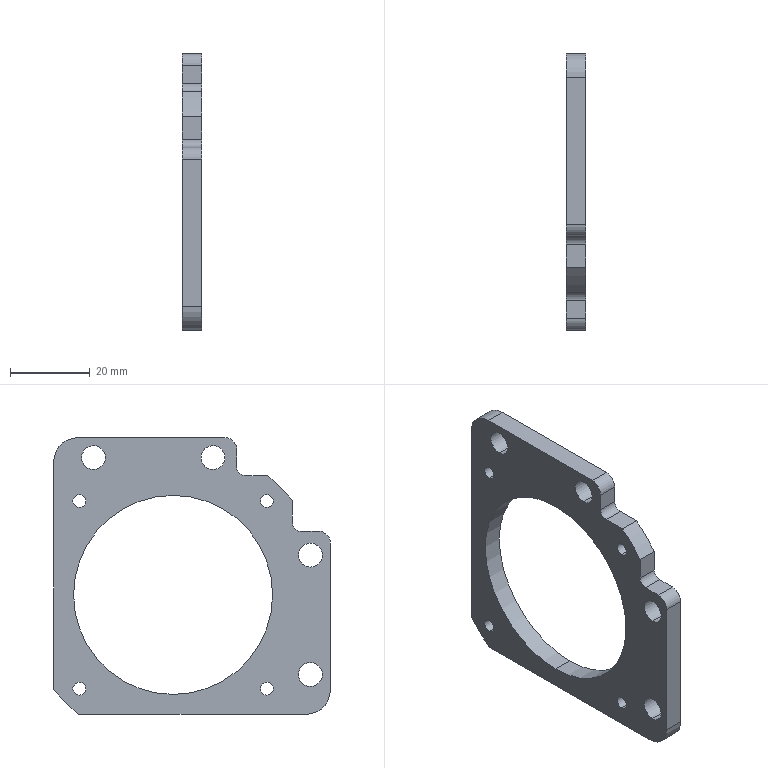CAM job | Mastercam | mm | 10 operations | part box 5 x 69.5 x 69.5
1. Facing | 20 - 63 平铣刀
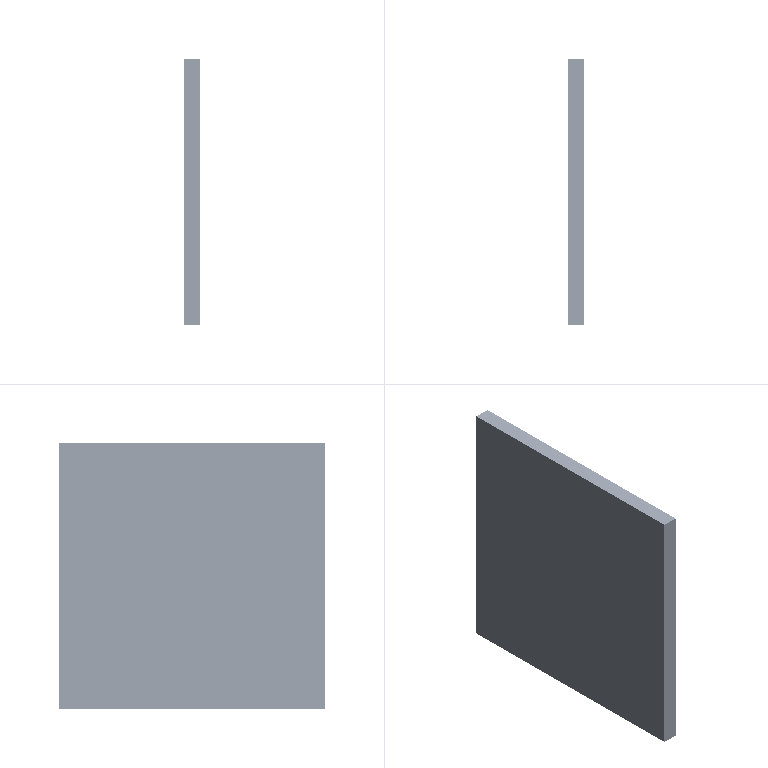2. 2D High Speed (2D Area Mill) | 8 - 8 平铣刀
3. 2D High Speed (2D Dynamic Mill) | 8 - 8 平铣刀
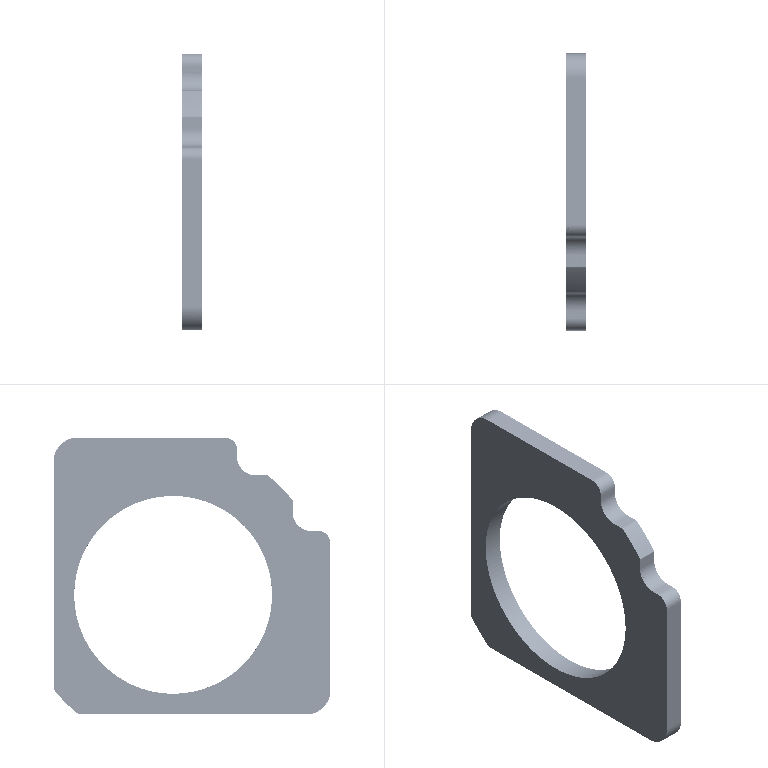4. Contour (Remachining) | 4 - 4 平铣刀
5. Contour (2D) | 4 - 4 平铣刀
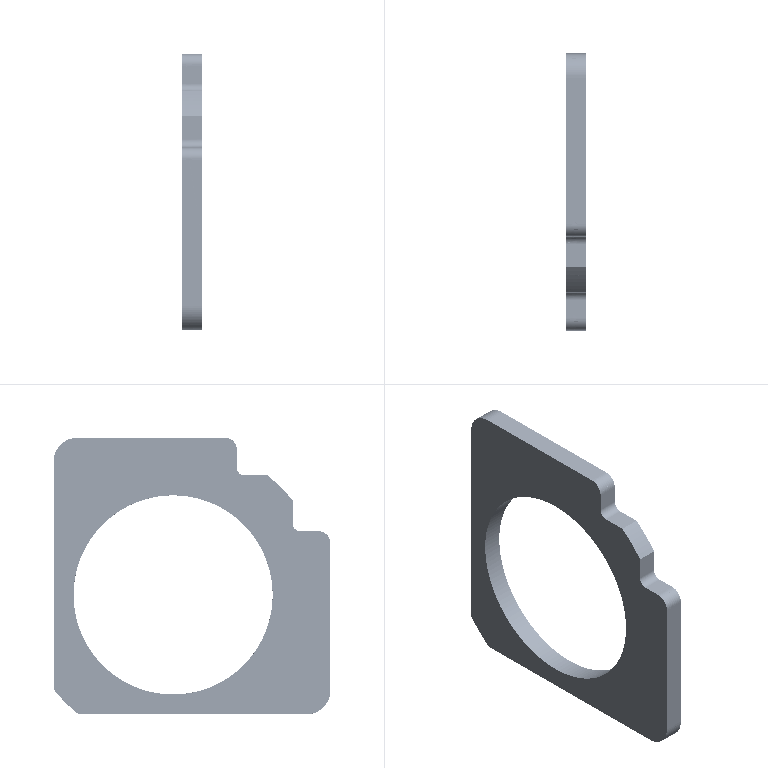6. Drill/Counterbore | 7 - 4 倒角刀
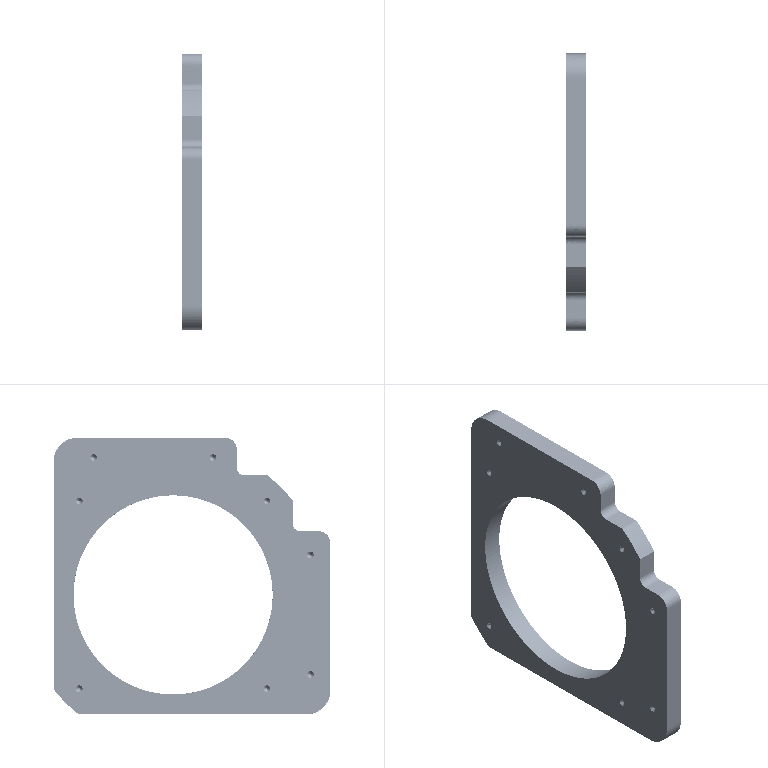7. Contour (2D chamfer) | 7 - 4 倒角刀
8. 2D High Speed (2D Dynamic Mill) | 8 - 8 平铣刀
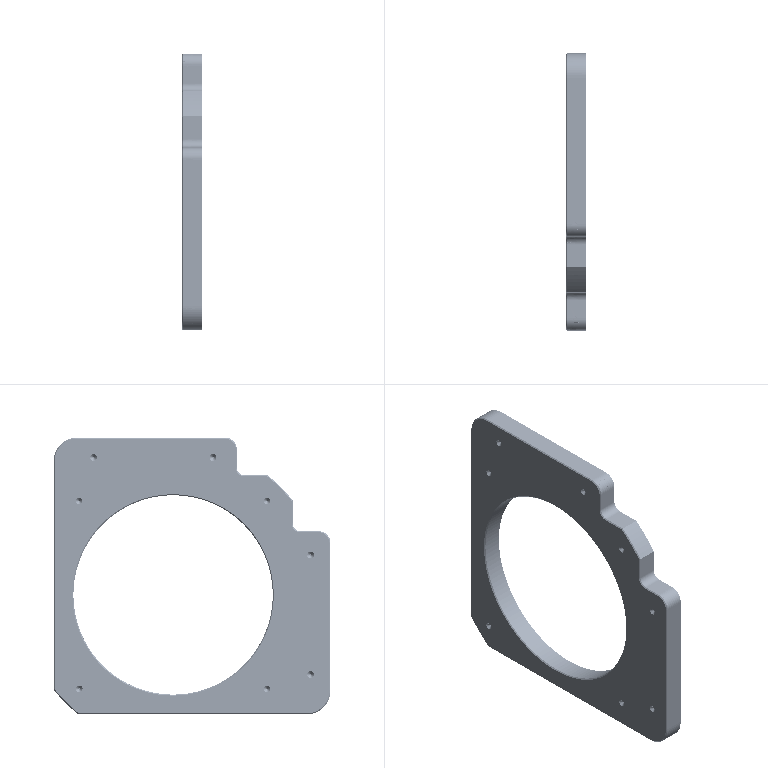9. Facing | 8 - 8 平铣刀
10. Contour (2D chamfer) | 7 - 4 倒角刀